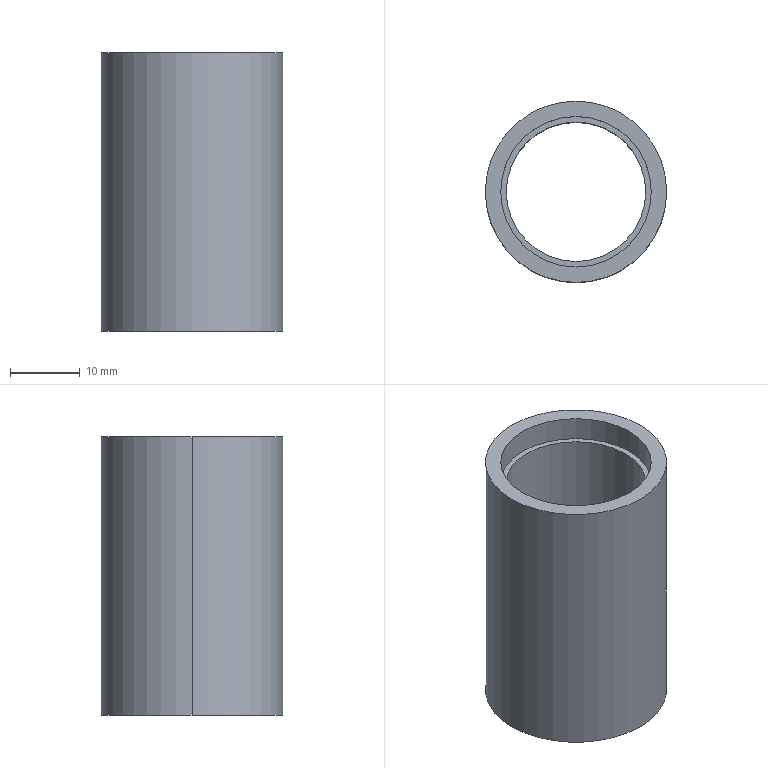Component | SolidWorks | RoundBarrel-1 | 1 solid | 12 faces | box 26 x 26 x 40 mm | volume 8305 mm3 | cylinder 8 | plane 4 | commonest cylinder face diameters 21.6 x4 26 x2 20 x2
build123d program:
from build123d import *

# Parameters (mm, degrees)
SKETCH1_2_R         = 13
SKETCH1_2_R_2       = 10
BOSS_EXTRUDE1_DEPTH = 40
SKETCH1_R           = 10.8
CUT_EXTRUDE1_DEPTH  = 3.5
CUT_EXTRUDE2_START  = -3.5
SKETCH2_R           = 10.8
CUT_EXTRUDE2_DEPTH  = 3.5


with BuildPart() as part:
    # Sketch1_2 → Boss-Extrude1 (new body)
    with BuildSketch(Plane.XY):
        Circle(SKETCH1_2_R)
        Circle(SKETCH1_2_R_2, mode=Mode.SUBTRACT)
    extrude(amount=BOSS_EXTRUDE1_DEPTH)

    # Sketch1 → Cut-Extrude1 (cut)
    with BuildSketch(Plane(origin=(0, 0, 0), x_dir=(-1, 0, 0), z_dir=(0, 0, -1))):
        Circle(SKETCH1_R)
    extrude(amount=-CUT_EXTRUDE1_DEPTH, mode=Mode.SUBTRACT)

    # Sketch2 → Cut-Extrude2 (cut)
    with BuildSketch(Plane.XY.offset(40).offset(CUT_EXTRUDE2_START)):
        with Locations(Location((0, 0, 0), (0, 0, 180))):
            Circle(SKETCH2_R)
    extrude(amount=CUT_EXTRUDE2_DEPTH, mode=Mode.SUBTRACT)


solid = part.part

# Placed as in the assembly
solid = solid.moved(Location((6.125, -1.646, 2.5), (0, 0, 0)))
STEP:
#1=COLOUR_RGB('',0.7922,0.8196,0.9333);
#2=FILL_AREA_STYLE_COLOUR('',#1);
#3=FILL_AREA_STYLE('',(#2));
#4=SURFACE_STYLE_FILL_AREA(#3);
#5=SURFACE_SIDE_STYLE('',(#4));
#6=SURFACE_STYLE_USAGE(.BOTH.,#5);
#7=PRESENTATION_STYLE_ASSIGNMENT((#6));
#8=CARTESIAN_POINT('',(-0.1841,-0.06482,1.535));
#9=VERTEX_POINT('',#8);
#10=CARTESIAN_POINT('',(0.6663,-0.06482,1.535));
#11=VERTEX_POINT('',#10);
#12=CARTESIAN_POINT('',(0.2411,-0.06482,1.535));
#13=DIRECTION('',(0.,0.,1.));
#14=DIRECTION('',(1.,0.,0.));
#15=AXIS2_PLACEMENT_3D('',#12,#13,#14);
#16=CIRCLE('',#15,0.4252);
#17=EDGE_CURVE('',#9,#11,#16,.T.);
#18=ORIENTED_EDGE('',*,*,#17,.F.);
#19=CARTESIAN_POINT('',(-0.1841,-0.06482,1.673));
#20=VERTEX_POINT('',#19);
#21=CARTESIAN_POINT('',(-0.1841,-0.06482,1.535));
#22=DIRECTION('',(0.,0.,1.));
#23=VECTOR('',#22,39.37);
#24=LINE('',#21,#23);
#25=EDGE_CURVE('',#9,#20,#24,.T.);
#26=ORIENTED_EDGE('',*,*,#25,.T.);
#27=CARTESIAN_POINT('',(0.6663,-0.06482,1.673));
#28=VERTEX_POINT('',#27);
#29=CARTESIAN_POINT('',(0.2411,-0.06482,1.673));
#30=DIRECTION('',(0.,0.,1.));
#31=DIRECTION('',(1.,0.,0.));
#32=AXIS2_PLACEMENT_3D('',#29,#30,#31);
#33=CIRCLE('',#32,0.4252);
#34=EDGE_CURVE('',#20,#28,#33,.T.);
#35=ORIENTED_EDGE('',*,*,#34,.T.);
#36=CARTESIAN_POINT('',(0.6663,-0.06482,1.535));
#37=DIRECTION('',(0.,0.,1.));
#38=VECTOR('',#37,39.37);
#39=LINE('',#36,#38);
#40=EDGE_CURVE('',#11,#28,#39,.T.);
#41=ORIENTED_EDGE('',*,*,#40,.F.);
#42=EDGE_LOOP('',(#18,#26,#35,#41));
#43=FACE_OUTER_BOUND('',#42,.T.);
#44=CARTESIAN_POINT('',(0.2411,-0.06482,1.535));
#45=DIRECTION('',(0.,0.,1.));
#46=DIRECTION('',(1.,0.,0.));
#47=AXIS2_PLACEMENT_3D('',#44,#45,#46);
#48=CYLINDRICAL_SURFACE('',#47,0.4252);
#49=ADVANCED_FACE('',(#43),#48,.F.);
#50=CARTESIAN_POINT('',(0.6663,-0.06482,0.2362));
#51=VERTEX_POINT('',#50);
#52=CARTESIAN_POINT('',(-0.1841,-0.06482,0.2362));
#53=VERTEX_POINT('',#52);
#54=CARTESIAN_POINT('',(0.2411,-0.06482,0.2362));
#55=DIRECTION('',(0.,0.,-1.));
#56=DIRECTION('',(-1.,0.,0.));
#57=AXIS2_PLACEMENT_3D('',#54,#55,#56);
#58=CIRCLE('',#57,0.4252);
#59=EDGE_CURVE('',#51,#53,#58,.T.);
#60=ORIENTED_EDGE('',*,*,#59,.F.);
#61=CARTESIAN_POINT('',(0.6663,-0.06482,0.09843));
#62=VERTEX_POINT('',#61);
#63=CARTESIAN_POINT('',(0.6663,-0.06482,0.2362));
#64=DIRECTION('',(0.,0.,-1.));
#65=VECTOR('',#64,39.37);
#66=LINE('',#63,#65);
#67=EDGE_CURVE('',#51,#62,#66,.T.);
#68=ORIENTED_EDGE('',*,*,#67,.T.);
#69=CARTESIAN_POINT('',(-0.1841,-0.06482,0.09843));
#70=VERTEX_POINT('',#69);
#71=CARTESIAN_POINT('',(0.2411,-0.06482,0.09843));
#72=DIRECTION('',(0.,0.,-1.));
#73=DIRECTION('',(-1.,0.,0.));
#74=AXIS2_PLACEMENT_3D('',#71,#72,#73);
#75=CIRCLE('',#74,0.4252);
#76=EDGE_CURVE('',#62,#70,#75,.T.);
#77=ORIENTED_EDGE('',*,*,#76,.T.);
#78=CARTESIAN_POINT('',(-0.1841,-0.06482,0.2362));
#79=DIRECTION('',(0.,0.,-1.));
#80=VECTOR('',#79,39.37);
#81=LINE('',#78,#80);
#82=EDGE_CURVE('',#53,#70,#81,.T.);
#83=ORIENTED_EDGE('',*,*,#82,.F.);
#84=EDGE_LOOP('',(#60,#68,#77,#83));
#85=FACE_OUTER_BOUND('',#84,.T.);
#86=CARTESIAN_POINT('',(0.2411,-0.06482,0.2362));
#87=DIRECTION('',(0.,0.,-1.));
#88=DIRECTION('',(-1.,0.,0.));
#89=AXIS2_PLACEMENT_3D('',#86,#87,#88);
#90=CYLINDRICAL_SURFACE('',#89,0.4252);
#91=ADVANCED_FACE('',(#85),#90,.F.);
#92=CARTESIAN_POINT('',(0.7529,-0.06482,1.673));
#93=VERTEX_POINT('',#92);
#94=CARTESIAN_POINT('',(-0.2707,-0.06482,1.673));
#95=VERTEX_POINT('',#94);
#96=CARTESIAN_POINT('',(0.2411,-0.06482,1.673));
#97=DIRECTION('',(0.,0.,1.));
#98=DIRECTION('',(1.,0.,0.));
#99=AXIS2_PLACEMENT_3D('',#96,#97,#98);
#100=CIRCLE('',#99,0.5118);
#101=EDGE_CURVE('',#93,#95,#100,.T.);
#102=ORIENTED_EDGE('',*,*,#101,.F.);
#103=CARTESIAN_POINT('',(0.7529,-0.06482,0.09843));
#104=VERTEX_POINT('',#103);
#105=CARTESIAN_POINT('',(0.7529,-0.06482,1.673));
#106=DIRECTION('',(0.,0.,-1.));
#107=VECTOR('',#106,39.37);
#108=LINE('',#105,#107);
#109=EDGE_CURVE('',#93,#104,#108,.T.);
#110=ORIENTED_EDGE('',*,*,#109,.T.);
#111=CARTESIAN_POINT('',(-0.2707,-0.06482,0.09843));
#112=VERTEX_POINT('',#111);
#113=CARTESIAN_POINT('',(0.2411,-0.06482,0.09843));
#114=DIRECTION('',(0.,0.,1.));
#115=DIRECTION('',(1.,0.,0.));
#116=AXIS2_PLACEMENT_3D('',#113,#114,#115);
#117=CIRCLE('',#116,0.5118);
#118=EDGE_CURVE('',#104,#112,#117,.T.);
#119=ORIENTED_EDGE('',*,*,#118,.T.);
#120=CARTESIAN_POINT('',(-0.2707,-0.06482,1.673));
#121=DIRECTION('',(0.,0.,-1.));
#122=VECTOR('',#121,39.37);
#123=LINE('',#120,#122);
#124=EDGE_CURVE('',#95,#112,#123,.T.);
#125=ORIENTED_EDGE('',*,*,#124,.F.);
#126=EDGE_LOOP('',(#102,#110,#119,#125));
#127=FACE_OUTER_BOUND('',#126,.T.);
#128=CARTESIAN_POINT('',(0.2411,-0.06482,1.673));
#129=DIRECTION('',(0.,0.,-1.));
#130=DIRECTION('',(-1.,0.,0.));
#131=AXIS2_PLACEMENT_3D('',#128,#129,#130);
#132=CYLINDRICAL_SURFACE('',#131,0.5118);
#133=ADVANCED_FACE('',(#127),#132,.T.);
#134=CARTESIAN_POINT('',(-0.1526,-0.06482,1.535));
#135=VERTEX_POINT('',#134);
#136=CARTESIAN_POINT('',(0.6348,-0.06482,1.535));
#137=VERTEX_POINT('',#136);
#138=CARTESIAN_POINT('',(0.2411,-0.06482,1.535));
#139=DIRECTION('',(0.,0.,1.));
#140=DIRECTION('',(1.,0.,0.));
#141=AXIS2_PLACEMENT_3D('',#138,#139,#140);
#142=CIRCLE('',#141,0.3937);
#143=EDGE_CURVE('',#135,#137,#142,.T.);
#144=ORIENTED_EDGE('',*,*,#143,.T.);
#145=CARTESIAN_POINT('',(0.6348,-0.06482,0.2362));
#146=VERTEX_POINT('',#145);
#147=CARTESIAN_POINT('',(0.6348,-0.06482,1.673));
#148=DIRECTION('',(0.,0.,-1.));
#149=VECTOR('',#148,39.37);
#150=LINE('',#147,#149);
#151=EDGE_CURVE('',#137,#146,#150,.T.);
#152=ORIENTED_EDGE('',*,*,#151,.T.);
#153=CARTESIAN_POINT('',(-0.1526,-0.06482,0.2362));
#154=VERTEX_POINT('',#153);
#155=CARTESIAN_POINT('',(0.2411,-0.06482,0.2362));
#156=DIRECTION('',(0.,0.,-1.));
#157=DIRECTION('',(-1.,0.,0.));
#158=AXIS2_PLACEMENT_3D('',#155,#156,#157);
#159=CIRCLE('',#158,0.3937);
#160=EDGE_CURVE('',#146,#154,#159,.T.);
#161=ORIENTED_EDGE('',*,*,#160,.T.);
#162=CARTESIAN_POINT('',(-0.1526,-0.06482,1.673));
#163=DIRECTION('',(0.,0.,-1.));
#164=VECTOR('',#163,39.37);
#165=LINE('',#162,#164);
#166=EDGE_CURVE('',#135,#154,#165,.T.);
#167=ORIENTED_EDGE('',*,*,#166,.F.);
#168=EDGE_LOOP('',(#144,#152,#161,#167));
#169=FACE_OUTER_BOUND('',#168,.T.);
#170=CARTESIAN_POINT('',(0.2411,-0.06482,1.673));
#171=DIRECTION('',(0.,0.,-1.));
#172=DIRECTION('',(-1.,0.,0.));
#173=AXIS2_PLACEMENT_3D('',#170,#171,#172);
#174=CYLINDRICAL_SURFACE('',#173,0.3937);
#175=ADVANCED_FACE('',(#169),#174,.F.);
#176=ORIENTED_EDGE('',*,*,#151,.F.);
#177=CARTESIAN_POINT('',(0.2411,-0.06482,1.535));
#178=DIRECTION('',(0.,0.,1.));
#179=DIRECTION('',(1.,0.,0.));
#180=AXIS2_PLACEMENT_3D('',#177,#178,#179);
#181=CIRCLE('',#180,0.3937);
#182=EDGE_CURVE('',#137,#135,#181,.T.);
#183=ORIENTED_EDGE('',*,*,#182,.T.);
#184=ORIENTED_EDGE('',*,*,#166,.T.);
#185=CARTESIAN_POINT('',(0.2411,-0.06482,0.2362));
#186=DIRECTION('',(0.,0.,-1.));
#187=DIRECTION('',(-1.,0.,0.));
#188=AXIS2_PLACEMENT_3D('',#185,#186,#187);
#189=CIRCLE('',#188,0.3937);
#190=EDGE_CURVE('',#154,#146,#189,.T.);
#191=ORIENTED_EDGE('',*,*,#190,.T.);
#192=EDGE_LOOP('',(#176,#183,#184,#191));
#193=FACE_OUTER_BOUND('',#192,.T.);
#194=CARTESIAN_POINT('',(0.2411,-0.06482,1.673));
#195=DIRECTION('',(0.,0.,-1.));
#196=DIRECTION('',(-1.,0.,0.));
#197=AXIS2_PLACEMENT_3D('',#194,#195,#196);
#198=CYLINDRICAL_SURFACE('',#197,0.3937);
#199=ADVANCED_FACE('',(#193),#198,.F.);
#200=CARTESIAN_POINT('',(0.2411,-0.06482,1.673));
#201=DIRECTION('',(0.,0.,1.));
#202=DIRECTION('',(1.,0.,0.));
#203=AXIS2_PLACEMENT_3D('',#200,#201,#202);
#204=CIRCLE('',#203,0.4252);
#205=EDGE_CURVE('',#28,#20,#204,.T.);
#206=ORIENTED_EDGE('',*,*,#205,.F.);
#207=ORIENTED_EDGE('',*,*,#34,.F.);
#208=EDGE_LOOP('',(#206,#207));
#209=FACE_BOUND('',#208,.T.);
#210=CARTESIAN_POINT('',(0.2411,-0.06482,1.673));
#211=DIRECTION('',(0.,0.,1.));
#212=DIRECTION('',(1.,0.,0.));
#213=AXIS2_PLACEMENT_3D('',#210,#211,#212);
#214=CIRCLE('',#213,0.5118);
#215=EDGE_CURVE('',#95,#93,#214,.T.);
#216=ORIENTED_EDGE('',*,*,#215,.T.);
#217=ORIENTED_EDGE('',*,*,#101,.T.);
#218=EDGE_LOOP('',(#216,#217));
#219=FACE_OUTER_BOUND('',#218,.T.);
#220=CARTESIAN_POINT('',(0.2411,-0.06482,1.673));
#221=DIRECTION('',(0.,0.,1.));
#222=DIRECTION('',(1.,0.,0.));
#223=AXIS2_PLACEMENT_3D('',#220,#221,#222);
#224=PLANE('',#223);
#225=ADVANCED_FACE('',(#209,#219),#224,.T.);
#226=CARTESIAN_POINT('',(0.2411,-0.06482,0.09843));
#227=DIRECTION('',(0.,0.,-1.));
#228=DIRECTION('',(-1.,0.,0.));
#229=AXIS2_PLACEMENT_3D('',#226,#227,#228);
#230=CIRCLE('',#229,0.4252);
#231=EDGE_CURVE('',#70,#62,#230,.T.);
#232=ORIENTED_EDGE('',*,*,#231,.F.);
#233=ORIENTED_EDGE('',*,*,#76,.F.);
#234=EDGE_LOOP('',(#232,#233));
#235=FACE_BOUND('',#234,.T.);
#236=CARTESIAN_POINT('',(0.2411,-0.06482,0.09843));
#237=DIRECTION('',(0.,0.,1.));
#238=DIRECTION('',(1.,0.,0.));
#239=AXIS2_PLACEMENT_3D('',#236,#237,#238);
#240=CIRCLE('',#239,0.5118);
#241=EDGE_CURVE('',#112,#104,#240,.T.);
#242=ORIENTED_EDGE('',*,*,#241,.F.);
#243=ORIENTED_EDGE('',*,*,#118,.F.);
#244=EDGE_LOOP('',(#242,#243));
#245=FACE_OUTER_BOUND('',#244,.T.);
#246=CARTESIAN_POINT('',(0.2411,-0.06482,0.09843));
#247=DIRECTION('',(0.,0.,1.));
#248=DIRECTION('',(1.,0.,0.));
#249=AXIS2_PLACEMENT_3D('',#246,#247,#248);
#250=PLANE('',#249);
#251=ADVANCED_FACE('',(#235,#245),#250,.F.);
#252=ORIENTED_EDGE('',*,*,#109,.F.);
#253=ORIENTED_EDGE('',*,*,#215,.F.);
#254=ORIENTED_EDGE('',*,*,#124,.T.);
#255=ORIENTED_EDGE('',*,*,#241,.T.);
#256=EDGE_LOOP('',(#252,#253,#254,#255));
#257=FACE_OUTER_BOUND('',#256,.T.);
#258=CARTESIAN_POINT('',(0.2411,-0.06482,1.673));
#259=DIRECTION('',(0.,0.,-1.));
#260=DIRECTION('',(-1.,0.,0.));
#261=AXIS2_PLACEMENT_3D('',#258,#259,#260);
#262=CYLINDRICAL_SURFACE('',#261,0.5118);
#263=ADVANCED_FACE('',(#257),#262,.T.);
#264=ORIENTED_EDGE('',*,*,#67,.F.);
#265=CARTESIAN_POINT('',(0.2411,-0.06482,0.2362));
#266=DIRECTION('',(0.,0.,-1.));
#267=DIRECTION('',(-1.,0.,0.));
#268=AXIS2_PLACEMENT_3D('',#265,#266,#267);
#269=CIRCLE('',#268,0.4252);
#270=EDGE_CURVE('',#53,#51,#269,.T.);
#271=ORIENTED_EDGE('',*,*,#270,.F.);
#272=ORIENTED_EDGE('',*,*,#82,.T.);
#273=ORIENTED_EDGE('',*,*,#231,.T.);
#274=EDGE_LOOP('',(#264,#271,#272,#273));
#275=FACE_OUTER_BOUND('',#274,.T.);
#276=CARTESIAN_POINT('',(0.2411,-0.06482,0.2362));
#277=DIRECTION('',(0.,0.,-1.));
#278=DIRECTION('',(-1.,0.,0.));
#279=AXIS2_PLACEMENT_3D('',#276,#277,#278);
#280=CYLINDRICAL_SURFACE('',#279,0.4252);
#281=ADVANCED_FACE('',(#275),#280,.F.);
#282=ORIENTED_EDGE('',*,*,#190,.F.);
#283=ORIENTED_EDGE('',*,*,#160,.F.);
#284=EDGE_LOOP('',(#282,#283));
#285=FACE_BOUND('',#284,.T.);
#286=ORIENTED_EDGE('',*,*,#270,.T.);
#287=ORIENTED_EDGE('',*,*,#59,.T.);
#288=EDGE_LOOP('',(#286,#287));
#289=FACE_OUTER_BOUND('',#288,.T.);
#290=CARTESIAN_POINT('',(0.2411,-0.06482,0.2362));
#291=DIRECTION('',(0.,0.,-1.));
#292=DIRECTION('',(-1.,0.,0.));
#293=AXIS2_PLACEMENT_3D('',#290,#291,#292);
#294=PLANE('',#293);
#295=ADVANCED_FACE('',(#285,#289),#294,.T.);
#296=ORIENTED_EDGE('',*,*,#25,.F.);
#297=CARTESIAN_POINT('',(0.2411,-0.06482,1.535));
#298=DIRECTION('',(0.,0.,1.));
#299=DIRECTION('',(1.,0.,0.));
#300=AXIS2_PLACEMENT_3D('',#297,#298,#299);
#301=CIRCLE('',#300,0.4252);
#302=EDGE_CURVE('',#11,#9,#301,.T.);
#303=ORIENTED_EDGE('',*,*,#302,.F.);
#304=ORIENTED_EDGE('',*,*,#40,.T.);
#305=ORIENTED_EDGE('',*,*,#205,.T.);
#306=EDGE_LOOP('',(#296,#303,#304,#305));
#307=FACE_OUTER_BOUND('',#306,.T.);
#308=CARTESIAN_POINT('',(0.2411,-0.06482,1.535));
#309=DIRECTION('',(0.,0.,1.));
#310=DIRECTION('',(1.,0.,0.));
#311=AXIS2_PLACEMENT_3D('',#308,#309,#310);
#312=CYLINDRICAL_SURFACE('',#311,0.4252);
#313=ADVANCED_FACE('',(#307),#312,.F.);
#314=ORIENTED_EDGE('',*,*,#143,.F.);
#315=ORIENTED_EDGE('',*,*,#182,.F.);
#316=EDGE_LOOP('',(#314,#315));
#317=FACE_BOUND('',#316,.T.);
#318=ORIENTED_EDGE('',*,*,#302,.T.);
#319=ORIENTED_EDGE('',*,*,#17,.T.);
#320=EDGE_LOOP('',(#318,#319));
#321=FACE_OUTER_BOUND('',#320,.T.);
#322=CARTESIAN_POINT('',(0.2411,-0.06482,1.535));
#323=DIRECTION('',(0.,0.,1.));
#324=DIRECTION('',(1.,0.,0.));
#325=AXIS2_PLACEMENT_3D('',#322,#323,#324);
#326=PLANE('',#325);
#327=ADVANCED_FACE('',(#317,#321),#326,.T.);
#328=CLOSED_SHELL('',(#49,#91,#133,#175,#199,#225,#251,#263,#281,#295,#313,#327));
#329=MANIFOLD_SOLID_BREP('',#328);
#330=STYLED_ITEM('',(#7),#329);
#331=(LENGTH_UNIT()NAMED_UNIT(*)SI_UNIT($,.METRE.));
#332=LENGTH_MEASURE_WITH_UNIT(LENGTH_MEASURE(0.0254),#331);
#333=DIMENSIONAL_EXPONENTS(1.,0.,0.,0.,0.,0.,0.);
#334=(CONVERSION_BASED_UNIT('',#332)LENGTH_UNIT()NAMED_UNIT(#333));
#335=UNCERTAINTY_MEASURE_WITH_UNIT(LENGTH_MEASURE(0.00001),#334,'','');
#336=(NAMED_UNIT(*)PLANE_ANGLE_UNIT()SI_UNIT($,.RADIAN.));
#337=(NAMED_UNIT(*)SI_UNIT($,.STERADIAN.)SOLID_ANGLE_UNIT());
#338=(GEOMETRIC_REPRESENTATION_CONTEXT(3)GLOBAL_UNCERTAINTY_ASSIGNED_CONTEXT((#335))GLOBAL_UNIT_ASSIGNED_CONTEXT((#334,#336,#337))REPRESENTATION_CONTEXT('',''));
#339=MECHANICAL_DESIGN_GEOMETRIC_PRESENTATION_REPRESENTATION('',(#330),#338);
#340=PRESENTATION_LAYER_ASSIGNMENT('','',(#330));
#341=CARTESIAN_POINT('',(0.,0.,0.));
#342=DIRECTION('',(0.,0.,1.));
#343=DIRECTION('',(1.,0.,0.));
#344=AXIS2_PLACEMENT_3D('',#341,#342,#343);
#345=(LENGTH_UNIT()NAMED_UNIT(*)SI_UNIT($,.METRE.));
#346=LENGTH_MEASURE_WITH_UNIT(LENGTH_MEASURE(0.0254),#345);
#347=DIMENSIONAL_EXPONENTS(1.,0.,0.,0.,0.,0.,0.);
#348=(CONVERSION_BASED_UNIT('',#346)LENGTH_UNIT()NAMED_UNIT(#347));
#349=UNCERTAINTY_MEASURE_WITH_UNIT(LENGTH_MEASURE(0.00001),#348,'','');
#350=(NAMED_UNIT(*)PLANE_ANGLE_UNIT()SI_UNIT($,.RADIAN.));
#351=(NAMED_UNIT(*)SI_UNIT($,.STERADIAN.)SOLID_ANGLE_UNIT());
#352=(GEOMETRIC_REPRESENTATION_CONTEXT(3)GLOBAL_UNCERTAINTY_ASSIGNED_CONTEXT((#349))GLOBAL_UNIT_ASSIGNED_CONTEXT((#348,#350,#351))REPRESENTATION_CONTEXT('',''));
#353=ADVANCED_BREP_SHAPE_REPRESENTATION('',(#329,#344),#352);